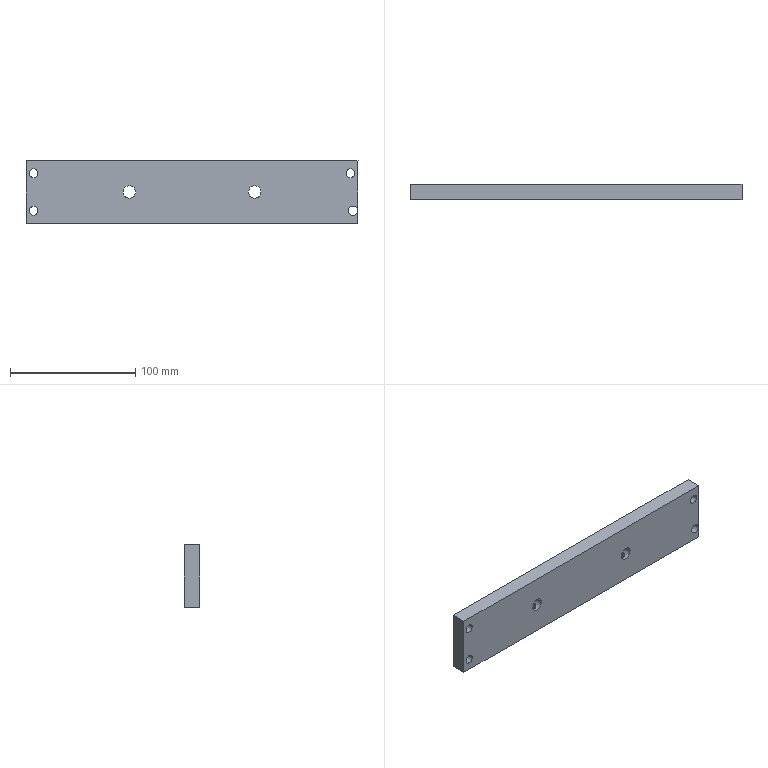Component | SolidWorks | AdjustmentTopPlate-1 | 1 solid | 22 faces | box 265 x 12 x 50 mm | volume 153730 mm3 | cylinder 16 | plane 6 | commonest cylinder face diameters 7 x6 6.8 x4 10 x4 7.46 x2
build123d program:
from build123d import *

# Parameters (mm, degrees)
SKETCH1_W             = 265
SKETCH1_H             = 50
SKETCH1_R             = 3.5
SKETCH1_R_2           = 3.73
EXTRUDE1_DEPTH        = 12
SKETCH2_R             = 5
EXTRUDE2_DEPTH        = 252.765
M8_TAPPED_HOLE1_D     = 6.8
M8_TAPPED_HOLE1_DEPTH = 22.25
M8_TAPPED_HOLE1_TIP   = 2.043


with BuildPart() as part:
    # Sketch1 → Extrude1 (new body)
    with BuildSketch(Plane.XY):
        with Locations((115.517, -16.583)):
            Rectangle(SKETCH1_W, SKETCH1_H)
        with Locations((-10.983, -1.583)):
            Circle(SKETCH1_R, mode=Mode.SUBTRACT)
        with Locations((242.017, -1.649)):
            Circle(SKETCH1_R, mode=Mode.SUBTRACT)
        with Locations((-10.983, -31.583)):
            Circle(SKETCH1_R, mode=Mode.SUBTRACT)
        with Locations((244.017, -31.583)):
            Circle(SKETCH1_R_2, mode=Mode.SUBTRACT)
    extrude(amount=EXTRUDE1_DEPTH)

    # Sketch2 → Extrude2 (cut, through all)
    with BuildSketch(Plane.XY.offset(12)):
        with Locations((65.517, -16.583)):
            Circle(SKETCH2_R)
        with Locations((165.517, -16.583)):
            Circle(SKETCH2_R)
    extrude(amount=-EXTRUDE2_DEPTH, mode=Mode.SUBTRACT)

    # M8 Tapped Hole1
    with Locations(Plane.XZ.offset(41.583)):
        with Locations((65.517, 6), (165.517, 6)):
            Hole(M8_TAPPED_HOLE1_D / 2, depth=M8_TAPPED_HOLE1_DEPTH)
            with Locations((0, 0, -(M8_TAPPED_HOLE1_DEPTH + M8_TAPPED_HOLE1_TIP / 2))):  # 118° drill point
                Cone(0, M8_TAPPED_HOLE1_D / 2, M8_TAPPED_HOLE1_TIP, mode=Mode.SUBTRACT)


solid = part.part

# Placed as in the assembly
solid = solid.moved(Location((-280.301, 717.983, -63.917), (90, 0, 0)))
STEP:
#1=CARTESIAN_POINT('',(-8.456,27.897,-3.366));
#2=VERTEX_POINT('',#1);
#3=CARTESIAN_POINT('',(-8.456,28.165,-3.366));
#4=VERTEX_POINT('',#3);
#5=CARTESIAN_POINT('',(-8.456,27.897,-3.366));
#6=CARTESIAN_POINT('',(-8.465,27.897,-3.366));
#7=CARTESIAN_POINT('',(-8.474,27.898,-3.366));
#8=CARTESIAN_POINT('',(-8.492,27.902,-3.363));
#9=CARTESIAN_POINT('',(-8.5,27.904,-3.361));
#10=CARTESIAN_POINT('',(-8.517,27.911,-3.357));
#11=CARTESIAN_POINT('',(-8.524,27.915,-3.354));
#12=CARTESIAN_POINT('',(-8.538,27.925,-3.348));
#13=CARTESIAN_POINT('',(-8.545,27.931,-3.345));
#14=CARTESIAN_POINT('',(-8.557,27.943,-3.338));
#15=CARTESIAN_POINT('',(-8.562,27.949,-3.335));
#16=CARTESIAN_POINT('',(-8.572,27.963,-3.329));
#17=CARTESIAN_POINT('',(-8.576,27.971,-3.325));
#18=CARTESIAN_POINT('',(-8.583,27.987,-3.32));
#19=CARTESIAN_POINT('',(-8.585,27.995,-3.318));
#20=CARTESIAN_POINT('',(-8.589,28.013,-3.314));
#21=CARTESIAN_POINT('',(-8.59,28.022,-3.314));
#22=CARTESIAN_POINT('',(-8.59,28.035,-3.314));
#23=CARTESIAN_POINT('',(-8.59,28.04,-3.314));
#24=CARTESIAN_POINT('',(-8.589,28.049,-3.315));
#25=CARTESIAN_POINT('',(-8.588,28.054,-3.315));
#26=CARTESIAN_POINT('',(-8.585,28.067,-3.318));
#27=CARTESIAN_POINT('',(-8.583,28.075,-3.32));
#28=CARTESIAN_POINT('',(-8.576,28.091,-3.326));
#29=CARTESIAN_POINT('',(-8.572,28.099,-3.329));
#30=CARTESIAN_POINT('',(-8.562,28.113,-3.335));
#31=CARTESIAN_POINT('',(-8.557,28.119,-3.338));
#32=CARTESIAN_POINT('',(-8.545,28.131,-3.345));
#33=CARTESIAN_POINT('',(-8.538,28.137,-3.348));
#34=CARTESIAN_POINT('',(-8.524,28.146,-3.354));
#35=CARTESIAN_POINT('',(-8.517,28.151,-3.357));
#36=CARTESIAN_POINT('',(-8.501,28.157,-3.361));
#37=CARTESIAN_POINT('',(-8.492,28.16,-3.363));
#38=CARTESIAN_POINT('',(-8.474,28.164,-3.366));
#39=CARTESIAN_POINT('',(-8.465,28.165,-3.366));
#40=CARTESIAN_POINT('',(-8.456,28.165,-3.366));
#41=B_SPLINE_CURVE_WITH_KNOTS('',3,(#5,#6,#7,#8,#9,#10,#11,#12,#13,#14,#15,#16,#17,#18,#19,#20,#21,#22,#23,#24,#25,#26,#27,#28,#29,#30,#31,#32,#33,#34,#35,#36,#37,#38,#39,#40),.UNSPECIFIED.,.F.,.F.,(4,2,2,2,2,2,2,2,2,2,2,2,2,2,2,2,2,4),(0.01101,0.0117,0.01239,0.01307,0.01376,0.01445,0.01513,0.01582,0.01651,0.01685,0.0172,0.01788,0.01857,0.01926,0.01995,0.02063,0.02132,0.02201),.UNSPECIFIED.);
#42=EDGE_CURVE('',#2,#4,#41,.T.);
#43=ORIENTED_EDGE('',*,*,#42,.F.);
#44=CARTESIAN_POINT('',(-8.456,27.897,-4.154));
#45=VERTEX_POINT('',#44);
#46=CARTESIAN_POINT('',(-8.456,27.897,-4.154));
#47=DIRECTION('',(-0.,-0.,-1.));
#48=VECTOR('',#47,39.37);
#49=LINE('',#46,#48);
#50=EDGE_CURVE('',#2,#45,#49,.T.);
#51=ORIENTED_EDGE('',*,*,#50,.T.);
#52=CARTESIAN_POINT('',(-8.456,28.165,-4.154));
#53=VERTEX_POINT('',#52);
#54=CARTESIAN_POINT('',(-8.456,28.031,-4.154));
#55=DIRECTION('',(-0.,-0.,-1.));
#56=DIRECTION('',(0.,1.,0.));
#57=AXIS2_PLACEMENT_3D('',#54,#55,#56);
#58=CIRCLE('',#57,0.1339);
#59=EDGE_CURVE('',#45,#53,#58,.T.);
#60=ORIENTED_EDGE('',*,*,#59,.T.);
#61=CARTESIAN_POINT('',(-8.456,28.165,-4.154));
#62=DIRECTION('',(-0.,-0.,-1.));
#63=VECTOR('',#62,39.37);
#64=LINE('',#61,#63);
#65=EDGE_CURVE('',#4,#53,#64,.T.);
#66=ORIENTED_EDGE('',*,*,#65,.F.);
#67=EDGE_LOOP('',(#43,#51,#60,#66));
#68=FACE_OUTER_BOUND('',#67,.T.);
#69=CARTESIAN_POINT('',(-8.456,28.031,-4.154));
#70=DIRECTION('',(-0.,-0.,-1.));
#71=DIRECTION('',(0.,1.,0.));
#72=AXIS2_PLACEMENT_3D('',#69,#70,#71);
#73=CYLINDRICAL_SURFACE('',#72,0.1339);
#74=ADVANCED_FACE('',(#68),#73,.F.);
#75=CARTESIAN_POINT('',(-4.519,27.897,-3.366));
#76=VERTEX_POINT('',#75);
#77=CARTESIAN_POINT('',(-4.519,28.165,-3.366));
#78=VERTEX_POINT('',#77);
#79=CARTESIAN_POINT('',(-4.519,27.897,-3.366));
#80=CARTESIAN_POINT('',(-4.528,27.897,-3.366));
#81=CARTESIAN_POINT('',(-4.537,27.898,-3.366));
#82=CARTESIAN_POINT('',(-4.555,27.902,-3.363));
#83=CARTESIAN_POINT('',(-4.563,27.904,-3.361));
#84=CARTESIAN_POINT('',(-4.58,27.911,-3.357));
#85=CARTESIAN_POINT('',(-4.587,27.915,-3.354));
#86=CARTESIAN_POINT('',(-4.601,27.925,-3.348));
#87=CARTESIAN_POINT('',(-4.608,27.931,-3.345));
#88=CARTESIAN_POINT('',(-4.62,27.943,-3.338));
#89=CARTESIAN_POINT('',(-4.625,27.949,-3.335));
#90=CARTESIAN_POINT('',(-4.635,27.963,-3.329));
#91=CARTESIAN_POINT('',(-4.639,27.971,-3.325));
#92=CARTESIAN_POINT('',(-4.646,27.987,-3.32));
#93=CARTESIAN_POINT('',(-4.648,27.995,-3.318));
#94=CARTESIAN_POINT('',(-4.652,28.013,-3.314));
#95=CARTESIAN_POINT('',(-4.653,28.022,-3.314));
#96=CARTESIAN_POINT('',(-4.653,28.035,-3.314));
#97=CARTESIAN_POINT('',(-4.653,28.04,-3.314));
#98=CARTESIAN_POINT('',(-4.652,28.049,-3.315));
#99=CARTESIAN_POINT('',(-4.651,28.054,-3.315));
#100=CARTESIAN_POINT('',(-4.648,28.067,-3.318));
#101=CARTESIAN_POINT('',(-4.646,28.075,-3.32));
#102=CARTESIAN_POINT('',(-4.639,28.091,-3.326));
#103=CARTESIAN_POINT('',(-4.635,28.099,-3.329));
#104=CARTESIAN_POINT('',(-4.625,28.113,-3.335));
#105=CARTESIAN_POINT('',(-4.62,28.119,-3.338));
#106=CARTESIAN_POINT('',(-4.608,28.131,-3.345));
#107=CARTESIAN_POINT('',(-4.601,28.137,-3.348));
#108=CARTESIAN_POINT('',(-4.587,28.146,-3.354));
#109=CARTESIAN_POINT('',(-4.58,28.151,-3.357));
#110=CARTESIAN_POINT('',(-4.564,28.157,-3.361));
#111=CARTESIAN_POINT('',(-4.555,28.16,-3.363));
#112=CARTESIAN_POINT('',(-4.537,28.164,-3.366));
#113=CARTESIAN_POINT('',(-4.528,28.165,-3.366));
#114=CARTESIAN_POINT('',(-4.519,28.165,-3.366));
#115=B_SPLINE_CURVE_WITH_KNOTS('',3,(#79,#80,#81,#82,#83,#84,#85,#86,#87,#88,#89,#90,#91,#92,#93,#94,#95,#96,#97,#98,#99,#100,#101,#102,#103,#104,#105,#106,#107,#108,#109,#110,#111,#112,#113,#114),.UNSPECIFIED.,.F.,.F.,(4,2,2,2,2,2,2,2,2,2,2,2,2,2,2,2,2,4),(0.01101,0.0117,0.01239,0.01307,0.01376,0.01445,0.01513,0.01582,0.01651,0.01685,0.0172,0.01788,0.01857,0.01926,0.01995,0.02063,0.02132,0.02201),.UNSPECIFIED.);
#116=EDGE_CURVE('',#76,#78,#115,.T.);
#117=ORIENTED_EDGE('',*,*,#116,.F.);
#118=CARTESIAN_POINT('',(-4.519,27.897,-4.154));
#119=VERTEX_POINT('',#118);
#120=CARTESIAN_POINT('',(-4.519,27.897,-4.154));
#121=DIRECTION('',(-0.,-0.,-1.));
#122=VECTOR('',#121,39.37);
#123=LINE('',#120,#122);
#124=EDGE_CURVE('',#76,#119,#123,.T.);
#125=ORIENTED_EDGE('',*,*,#124,.T.);
#126=CARTESIAN_POINT('',(-4.519,28.165,-4.154));
#127=VERTEX_POINT('',#126);
#128=CARTESIAN_POINT('',(-4.519,28.031,-4.154));
#129=DIRECTION('',(-0.,-0.,-1.));
#130=DIRECTION('',(0.,1.,0.));
#131=AXIS2_PLACEMENT_3D('',#128,#129,#130);
#132=CIRCLE('',#131,0.1339);
#133=EDGE_CURVE('',#119,#127,#132,.T.);
#134=ORIENTED_EDGE('',*,*,#133,.T.);
#135=CARTESIAN_POINT('',(-4.519,28.165,-4.154));
#136=DIRECTION('',(-0.,-0.,-1.));
#137=VECTOR('',#136,39.37);
#138=LINE('',#135,#137);
#139=EDGE_CURVE('',#78,#127,#138,.T.);
#140=ORIENTED_EDGE('',*,*,#139,.F.);
#141=EDGE_LOOP('',(#117,#125,#134,#140));
#142=FACE_OUTER_BOUND('',#141,.T.);
#143=CARTESIAN_POINT('',(-4.519,28.031,-4.154));
#144=DIRECTION('',(-0.,-0.,-1.));
#145=DIRECTION('',(0.,1.,0.));
#146=AXIS2_PLACEMENT_3D('',#143,#144,#145);
#147=CYLINDRICAL_SURFACE('',#146,0.1339);
#148=ADVANCED_FACE('',(#142),#147,.F.);
#149=CARTESIAN_POINT('',(-4.519,28.165,-3.366));
#150=CARTESIAN_POINT('',(-4.51,28.165,-3.366));
#151=CARTESIAN_POINT('',(-4.501,28.164,-3.366));
#152=CARTESIAN_POINT('',(-4.483,28.16,-3.363));
#153=CARTESIAN_POINT('',(-4.475,28.157,-3.361));
#154=CARTESIAN_POINT('',(-4.459,28.151,-3.357));
#155=CARTESIAN_POINT('',(-4.451,28.146,-3.354));
#156=CARTESIAN_POINT('',(-4.437,28.137,-3.348));
#157=CARTESIAN_POINT('',(-4.43,28.131,-3.345));
#158=CARTESIAN_POINT('',(-4.418,28.119,-3.338));
#159=CARTESIAN_POINT('',(-4.413,28.113,-3.335));
#160=CARTESIAN_POINT('',(-4.403,28.099,-3.329));
#161=CARTESIAN_POINT('',(-4.399,28.091,-3.326));
#162=CARTESIAN_POINT('',(-4.392,28.075,-3.32));
#163=CARTESIAN_POINT('',(-4.39,28.067,-3.318));
#164=CARTESIAN_POINT('',(-4.387,28.054,-3.315));
#165=CARTESIAN_POINT('',(-4.386,28.049,-3.315));
#166=CARTESIAN_POINT('',(-4.385,28.04,-3.314));
#167=CARTESIAN_POINT('',(-4.385,28.035,-3.314));
#168=CARTESIAN_POINT('',(-4.385,28.022,-3.314));
#169=CARTESIAN_POINT('',(-4.386,28.013,-3.314));
#170=CARTESIAN_POINT('',(-4.39,27.995,-3.318));
#171=CARTESIAN_POINT('',(-4.392,27.987,-3.32));
#172=CARTESIAN_POINT('',(-4.399,27.971,-3.325));
#173=CARTESIAN_POINT('',(-4.403,27.963,-3.329));
#174=CARTESIAN_POINT('',(-4.413,27.949,-3.335));
#175=CARTESIAN_POINT('',(-4.418,27.943,-3.338));
#176=CARTESIAN_POINT('',(-4.436,27.924,-3.348));
#177=CARTESIAN_POINT('',(-4.45,27.915,-3.354));
#178=CARTESIAN_POINT('',(-4.475,27.904,-3.361));
#179=CARTESIAN_POINT('',(-4.483,27.902,-3.363));
#180=CARTESIAN_POINT('',(-4.501,27.898,-3.365));
#181=CARTESIAN_POINT('',(-4.51,27.897,-3.366));
#182=CARTESIAN_POINT('',(-4.519,27.897,-3.366));
#183=B_SPLINE_CURVE_WITH_KNOTS('',3,(#149,#150,#151,#152,#153,#154,#155,#156,#157,#158,#159,#160,#161,#162,#163,#164,#165,#166,#167,#168,#169,#170,#171,#172,#173,#174,#175,#176,#177,#178,#179,#180,#181,#182),.UNSPECIFIED.,.F.,.F.,(4,2,2,2,2,2,2,2,2,2,2,2,2,2,2,2,4),(0.,0.0006882,0.001376,0.002065,0.002753,0.003441,0.004129,0.004818,0.005162,0.005506,0.006194,0.006882,0.007571,0.008259,0.009635,0.01032,0.01101),.UNSPECIFIED.);
#184=EDGE_CURVE('',#78,#76,#183,.T.);
#185=ORIENTED_EDGE('',*,*,#184,.T.);
#186=ORIENTED_EDGE('',*,*,#116,.T.);
#187=EDGE_LOOP('',(#185,#186));
#188=FACE_BOUND('',#187,.T.);
#189=CARTESIAN_POINT('',(-4.716,28.267,-3.169));
#190=VERTEX_POINT('',#189);
#191=CARTESIAN_POINT('',(-4.322,28.267,-3.169));
#192=VERTEX_POINT('',#191);
#193=CARTESIAN_POINT('',(-4.519,28.267,-3.169));
#194=DIRECTION('',(0.,-1.,0.));
#195=DIRECTION('',(1.,0.,-0.));
#196=AXIS2_PLACEMENT_3D('',#193,#194,#195);
#197=CIRCLE('',#196,0.1969);
#198=EDGE_CURVE('',#190,#192,#197,.T.);
#199=ORIENTED_EDGE('',*,*,#198,.F.);
#200=CARTESIAN_POINT('',(-4.716,27.795,-3.169));
#201=VERTEX_POINT('',#200);
#202=CARTESIAN_POINT('',(-4.716,28.267,-3.169));
#203=DIRECTION('',(0.,-1.,0.));
#204=VECTOR('',#203,39.37);
#205=LINE('',#202,#204);
#206=EDGE_CURVE('',#190,#201,#205,.T.);
#207=ORIENTED_EDGE('',*,*,#206,.T.);
#208=CARTESIAN_POINT('',(-4.322,27.795,-3.169));
#209=VERTEX_POINT('',#208);
#210=CARTESIAN_POINT('',(-4.519,27.795,-3.169));
#211=DIRECTION('',(0.,-1.,0.));
#212=DIRECTION('',(1.,0.,-0.));
#213=AXIS2_PLACEMENT_3D('',#210,#211,#212);
#214=CIRCLE('',#213,0.1969);
#215=EDGE_CURVE('',#201,#209,#214,.T.);
#216=ORIENTED_EDGE('',*,*,#215,.T.);
#217=CARTESIAN_POINT('',(-4.322,28.267,-3.169));
#218=DIRECTION('',(0.,-1.,0.));
#219=VECTOR('',#218,39.37);
#220=LINE('',#217,#219);
#221=EDGE_CURVE('',#192,#209,#220,.T.);
#222=ORIENTED_EDGE('',*,*,#221,.F.);
#223=EDGE_LOOP('',(#199,#207,#216,#222));
#224=FACE_OUTER_BOUND('',#223,.T.);
#225=CARTESIAN_POINT('',(-4.519,28.267,-3.169));
#226=DIRECTION('',(0.,-1.,0.));
#227=DIRECTION('',(1.,0.,-0.));
#228=AXIS2_PLACEMENT_3D('',#225,#226,#227);
#229=CYLINDRICAL_SURFACE('',#228,0.1969);
#230=ADVANCED_FACE('',(#188,#224),#229,.F.);
#231=CARTESIAN_POINT('',(-8.456,28.165,-3.366));
#232=CARTESIAN_POINT('',(-8.447,28.165,-3.366));
#233=CARTESIAN_POINT('',(-8.438,28.164,-3.366));
#234=CARTESIAN_POINT('',(-8.42,28.16,-3.363));
#235=CARTESIAN_POINT('',(-8.412,28.157,-3.361));
#236=CARTESIAN_POINT('',(-8.396,28.151,-3.357));
#237=CARTESIAN_POINT('',(-8.388,28.146,-3.354));
#238=CARTESIAN_POINT('',(-8.374,28.137,-3.348));
#239=CARTESIAN_POINT('',(-8.367,28.131,-3.345));
#240=CARTESIAN_POINT('',(-8.355,28.119,-3.338));
#241=CARTESIAN_POINT('',(-8.35,28.113,-3.335));
#242=CARTESIAN_POINT('',(-8.34,28.099,-3.329));
#243=CARTESIAN_POINT('',(-8.336,28.091,-3.326));
#244=CARTESIAN_POINT('',(-8.329,28.075,-3.32));
#245=CARTESIAN_POINT('',(-8.327,28.067,-3.318));
#246=CARTESIAN_POINT('',(-8.324,28.054,-3.315));
#247=CARTESIAN_POINT('',(-8.323,28.049,-3.315));
#248=CARTESIAN_POINT('',(-8.322,28.04,-3.314));
#249=CARTESIAN_POINT('',(-8.322,28.035,-3.314));
#250=CARTESIAN_POINT('',(-8.322,28.022,-3.314));
#251=CARTESIAN_POINT('',(-8.323,28.013,-3.314));
#252=CARTESIAN_POINT('',(-8.327,27.995,-3.318));
#253=CARTESIAN_POINT('',(-8.329,27.987,-3.32));
#254=CARTESIAN_POINT('',(-8.336,27.971,-3.325));
#255=CARTESIAN_POINT('',(-8.34,27.963,-3.329));
#256=CARTESIAN_POINT('',(-8.35,27.949,-3.335));
#257=CARTESIAN_POINT('',(-8.355,27.943,-3.338));
#258=CARTESIAN_POINT('',(-8.373,27.924,-3.348));
#259=CARTESIAN_POINT('',(-8.387,27.915,-3.354));
#260=CARTESIAN_POINT('',(-8.412,27.904,-3.361));
#261=CARTESIAN_POINT('',(-8.42,27.902,-3.363));
#262=CARTESIAN_POINT('',(-8.438,27.898,-3.365));
#263=CARTESIAN_POINT('',(-8.447,27.897,-3.366));
#264=CARTESIAN_POINT('',(-8.456,27.897,-3.366));
#265=B_SPLINE_CURVE_WITH_KNOTS('',3,(#231,#232,#233,#234,#235,#236,#237,#238,#239,#240,#241,#242,#243,#244,#245,#246,#247,#248,#249,#250,#251,#252,#253,#254,#255,#256,#257,#258,#259,#260,#261,#262,#263,#264),.UNSPECIFIED.,.F.,.F.,(4,2,2,2,2,2,2,2,2,2,2,2,2,2,2,2,4),(0.,0.0006882,0.001376,0.002065,0.002753,0.003441,0.004129,0.004818,0.005162,0.005506,0.006194,0.006882,0.007571,0.008259,0.009635,0.01032,0.01101),.UNSPECIFIED.);
#266=EDGE_CURVE('',#4,#2,#265,.T.);
#267=ORIENTED_EDGE('',*,*,#266,.T.);
#268=ORIENTED_EDGE('',*,*,#42,.T.);
#269=EDGE_LOOP('',(#267,#268));
#270=FACE_BOUND('',#269,.T.);
#271=CARTESIAN_POINT('',(-8.653,28.267,-3.169));
#272=VERTEX_POINT('',#271);
#273=CARTESIAN_POINT('',(-8.259,28.267,-3.169));
#274=VERTEX_POINT('',#273);
#275=CARTESIAN_POINT('',(-8.456,28.267,-3.169));
#276=DIRECTION('',(0.,-1.,0.));
#277=DIRECTION('',(1.,0.,-0.));
#278=AXIS2_PLACEMENT_3D('',#275,#276,#277);
#279=CIRCLE('',#278,0.1969);
#280=EDGE_CURVE('',#272,#274,#279,.T.);
#281=ORIENTED_EDGE('',*,*,#280,.F.);
#282=CARTESIAN_POINT('',(-8.653,27.795,-3.169));
#283=VERTEX_POINT('',#282);
#284=CARTESIAN_POINT('',(-8.653,28.267,-3.169));
#285=DIRECTION('',(0.,-1.,0.));
#286=VECTOR('',#285,39.37);
#287=LINE('',#284,#286);
#288=EDGE_CURVE('',#272,#283,#287,.T.);
#289=ORIENTED_EDGE('',*,*,#288,.T.);
#290=CARTESIAN_POINT('',(-8.259,27.795,-3.169));
#291=VERTEX_POINT('',#290);
#292=CARTESIAN_POINT('',(-8.456,27.795,-3.169));
#293=DIRECTION('',(0.,-1.,0.));
#294=DIRECTION('',(1.,0.,-0.));
#295=AXIS2_PLACEMENT_3D('',#292,#293,#294);
#296=CIRCLE('',#295,0.1969);
#297=EDGE_CURVE('',#283,#291,#296,.T.);
#298=ORIENTED_EDGE('',*,*,#297,.T.);
#299=CARTESIAN_POINT('',(-8.259,28.267,-3.169));
#300=DIRECTION('',(0.,-1.,0.));
#301=VECTOR('',#300,39.37);
#302=LINE('',#299,#301);
#303=EDGE_CURVE('',#274,#291,#302,.T.);
#304=ORIENTED_EDGE('',*,*,#303,.F.);
#305=EDGE_LOOP('',(#281,#289,#298,#304));
#306=FACE_OUTER_BOUND('',#305,.T.);
#307=CARTESIAN_POINT('',(-8.456,28.267,-3.169));
#308=DIRECTION('',(0.,-1.,0.));
#309=DIRECTION('',(1.,0.,-0.));
#310=AXIS2_PLACEMENT_3D('',#307,#308,#309);
#311=CYLINDRICAL_SURFACE('',#310,0.1969);
#312=ADVANCED_FACE('',(#270,#306),#311,.F.);
#313=CARTESIAN_POINT('',(-1.575,27.795,-3.76));
#314=VERTEX_POINT('',#313);
#315=CARTESIAN_POINT('',(-1.282,27.795,-3.76));
#316=VERTEX_POINT('',#315);
#317=CARTESIAN_POINT('',(-1.428,27.795,-3.76));
#318=DIRECTION('',(0.,-1.,0.));
#319=DIRECTION('',(1.,0.,-0.));
#320=AXIS2_PLACEMENT_3D('',#317,#318,#319);
#321=CIRCLE('',#320,0.1469);
#322=EDGE_CURVE('',#314,#316,#321,.T.);
#323=ORIENTED_EDGE('',*,*,#322,.T.);
#324=CARTESIAN_POINT('',(-1.282,28.267,-3.76));
#325=VERTEX_POINT('',#324);
#326=CARTESIAN_POINT('',(-1.282,27.795,-3.76));
#327=DIRECTION('',(-0.,1.,-0.));
#328=VECTOR('',#327,39.37);
#329=LINE('',#326,#328);
#330=EDGE_CURVE('',#316,#325,#329,.T.);
#331=ORIENTED_EDGE('',*,*,#330,.T.);
#332=CARTESIAN_POINT('',(-1.575,28.267,-3.76));
#333=VERTEX_POINT('',#332);
#334=CARTESIAN_POINT('',(-1.428,28.267,-3.76));
#335=DIRECTION('',(0.,-1.,0.));
#336=DIRECTION('',(1.,0.,-0.));
#337=AXIS2_PLACEMENT_3D('',#334,#335,#336);
#338=CIRCLE('',#337,0.1469);
#339=EDGE_CURVE('',#333,#325,#338,.T.);
#340=ORIENTED_EDGE('',*,*,#339,.F.);
#341=CARTESIAN_POINT('',(-1.575,27.795,-3.76));
#342=DIRECTION('',(-0.,1.,-0.));
#343=VECTOR('',#342,39.37);
#344=LINE('',#341,#343);
#345=EDGE_CURVE('',#314,#333,#344,.T.);
#346=ORIENTED_EDGE('',*,*,#345,.F.);
#347=EDGE_LOOP('',(#323,#331,#340,#346));
#348=FACE_OUTER_BOUND('',#347,.T.);
#349=CARTESIAN_POINT('',(-1.428,27.795,-3.76));
#350=DIRECTION('',(-0.,1.,-0.));
#351=DIRECTION('',(-1.,0.,0.));
#352=AXIS2_PLACEMENT_3D('',#349,#350,#351);
#353=CYLINDRICAL_SURFACE('',#352,0.1469);
#354=ADVANCED_FACE('',(#348),#353,.F.);
#355=CARTESIAN_POINT('',(-1.645,27.795,-2.581));
#356=VERTEX_POINT('',#355);
#357=CARTESIAN_POINT('',(-1.369,27.795,-2.581));
#358=VERTEX_POINT('',#357);
#359=CARTESIAN_POINT('',(-1.507,27.795,-2.581));
#360=DIRECTION('',(0.,-1.,0.));
#361=DIRECTION('',(1.,0.,-0.));
#362=AXIS2_PLACEMENT_3D('',#359,#360,#361);
#363=CIRCLE('',#362,0.1378);
#364=EDGE_CURVE('',#356,#358,#363,.T.);
#365=ORIENTED_EDGE('',*,*,#364,.T.);
#366=CARTESIAN_POINT('',(-1.369,28.267,-2.581));
#367=VERTEX_POINT('',#366);
#368=CARTESIAN_POINT('',(-1.369,27.795,-2.581));
#369=DIRECTION('',(-0.,1.,-0.));
#370=VECTOR('',#369,39.37);
#371=LINE('',#368,#370);
#372=EDGE_CURVE('',#358,#367,#371,.T.);
#373=ORIENTED_EDGE('',*,*,#372,.T.);
#374=CARTESIAN_POINT('',(-1.645,28.267,-2.581));
#375=VERTEX_POINT('',#374);
#376=CARTESIAN_POINT('',(-1.507,28.267,-2.581));
#377=DIRECTION('',(0.,-1.,0.));
#378=DIRECTION('',(1.,0.,-0.));
#379=AXIS2_PLACEMENT_3D('',#376,#377,#378);
#380=CIRCLE('',#379,0.1378);
#381=EDGE_CURVE('',#375,#367,#380,.T.);
#382=ORIENTED_EDGE('',*,*,#381,.F.);
#383=CARTESIAN_POINT('',(-1.645,27.795,-2.581));
#384=DIRECTION('',(-0.,1.,-0.));
#385=VECTOR('',#384,39.37);
#386=LINE('',#383,#385);
#387=EDGE_CURVE('',#356,#375,#386,.T.);
#388=ORIENTED_EDGE('',*,*,#387,.F.);
#389=EDGE_LOOP('',(#365,#373,#382,#388));
#390=FACE_OUTER_BOUND('',#389,.T.);
#391=CARTESIAN_POINT('',(-1.507,27.795,-2.581));
#392=DIRECTION('',(-0.,1.,-0.));
#393=DIRECTION('',(-1.,0.,0.));
#394=AXIS2_PLACEMENT_3D('',#391,#392,#393);
#395=CYLINDRICAL_SURFACE('',#394,0.1378);
#396=ADVANCED_FACE('',(#390),#395,.F.);
#397=CARTESIAN_POINT('',(-11.606,27.795,-2.579));
#398=VERTEX_POINT('',#397);
#399=CARTESIAN_POINT('',(-11.33,27.795,-2.579));
#400=VERTEX_POINT('',#399);
#401=CARTESIAN_POINT('',(-11.468,27.795,-2.579));
#402=DIRECTION('',(0.,-1.,0.));
#403=DIRECTION('',(1.,0.,-0.));
#404=AXIS2_PLACEMENT_3D('',#401,#402,#403);
#405=CIRCLE('',#404,0.1378);
#406=EDGE_CURVE('',#398,#400,#405,.T.);
#407=ORIENTED_EDGE('',*,*,#406,.T.);
#408=CARTESIAN_POINT('',(-11.33,28.267,-2.579));
#409=VERTEX_POINT('',#408);
#410=CARTESIAN_POINT('',(-11.33,27.795,-2.579));
#411=DIRECTION('',(-0.,1.,-0.));
#412=VECTOR('',#411,39.37);
#413=LINE('',#410,#412);
#414=EDGE_CURVE('',#400,#409,#413,.T.);
#415=ORIENTED_EDGE('',*,*,#414,.T.);
#416=CARTESIAN_POINT('',(-11.606,28.267,-2.579));
#417=VERTEX_POINT('',#416);
#418=CARTESIAN_POINT('',(-11.468,28.267,-2.579));
#419=DIRECTION('',(0.,-1.,0.));
#420=DIRECTION('',(1.,0.,-0.));
#421=AXIS2_PLACEMENT_3D('',#418,#419,#420);
#422=CIRCLE('',#421,0.1378);
#423=EDGE_CURVE('',#417,#409,#422,.T.);
#424=ORIENTED_EDGE('',*,*,#423,.F.);
#425=CARTESIAN_POINT('',(-11.606,27.795,-2.579));
#426=DIRECTION('',(-0.,1.,-0.));
#427=VECTOR('',#426,39.37);
#428=LINE('',#425,#427);
#429=EDGE_CURVE('',#398,#417,#428,.T.);
#430=ORIENTED_EDGE('',*,*,#429,.F.);
#431=EDGE_LOOP('',(#407,#415,#424,#430));
#432=FACE_OUTER_BOUND('',#431,.T.);
#433=CARTESIAN_POINT('',(-11.468,27.795,-2.579));
#434=DIRECTION('',(-0.,1.,-0.));
#435=DIRECTION('',(-1.,0.,0.));
#436=AXIS2_PLACEMENT_3D('',#433,#434,#435);
#437=CYLINDRICAL_SURFACE('',#436,0.1378);
#438=ADVANCED_FACE('',(#432),#437,.F.);
#439=CARTESIAN_POINT('',(-11.606,27.795,-3.76));
#440=VERTEX_POINT('',#439);
#441=CARTESIAN_POINT('',(-11.33,27.795,-3.76));
#442=VERTEX_POINT('',#441);
#443=CARTESIAN_POINT('',(-11.468,27.795,-3.76));
#444=DIRECTION('',(0.,-1.,0.));
#445=DIRECTION('',(1.,0.,-0.));
#446=AXIS2_PLACEMENT_3D('',#443,#444,#445);
#447=CIRCLE('',#446,0.1378);
#448=EDGE_CURVE('',#440,#442,#447,.T.);
#449=ORIENTED_EDGE('',*,*,#448,.T.);
#450=CARTESIAN_POINT('',(-11.33,28.267,-3.76));
#451=VERTEX_POINT('',#450);
#452=CARTESIAN_POINT('',(-11.33,27.795,-3.76));
#453=DIRECTION('',(-0.,1.,-0.));
#454=VECTOR('',#453,39.37);
#455=LINE('',#452,#454);
#456=EDGE_CURVE('',#442,#451,#455,.T.);
#457=ORIENTED_EDGE('',*,*,#456,.T.);
#458=CARTESIAN_POINT('',(-11.606,28.267,-3.76));
#459=VERTEX_POINT('',#458);
#460=CARTESIAN_POINT('',(-11.468,28.267,-3.76));
#461=DIRECTION('',(0.,-1.,0.));
#462=DIRECTION('',(1.,0.,-0.));
#463=AXIS2_PLACEMENT_3D('',#460,#461,#462);
#464=CIRCLE('',#463,0.1378);
#465=EDGE_CURVE('',#459,#451,#464,.T.);
#466=ORIENTED_EDGE('',*,*,#465,.F.);
#467=CARTESIAN_POINT('',(-11.606,27.795,-3.76));
#468=DIRECTION('',(-0.,1.,-0.));
#469=VECTOR('',#468,39.37);
#470=LINE('',#467,#469);
#471=EDGE_CURVE('',#440,#459,#470,.T.);
#472=ORIENTED_EDGE('',*,*,#471,.F.);
#473=EDGE_LOOP('',(#449,#457,#466,#472));
#474=FACE_OUTER_BOUND('',#473,.T.);
#475=CARTESIAN_POINT('',(-11.468,27.795,-3.76));
#476=DIRECTION('',(-0.,1.,-0.));
#477=DIRECTION('',(-1.,0.,0.));
#478=AXIS2_PLACEMENT_3D('',#475,#476,#477);
#479=CYLINDRICAL_SURFACE('',#478,0.1378);
#480=ADVANCED_FACE('',(#474),#479,.F.);
#481=CARTESIAN_POINT('',(-4.519,27.795,-3.169));
#482=DIRECTION('',(0.,-1.,0.));
#483=DIRECTION('',(1.,0.,-0.));
#484=AXIS2_PLACEMENT_3D('',#481,#482,#483);
#485=CIRCLE('',#484,0.1969);
#486=EDGE_CURVE('',#209,#201,#485,.T.);
#487=ORIENTED_EDGE('',*,*,#486,.F.);
#488=ORIENTED_EDGE('',*,*,#215,.F.);
#489=EDGE_LOOP('',(#487,#488));
#490=FACE_BOUND('',#489,.T.);
#491=CARTESIAN_POINT('',(-8.456,27.795,-3.169));
#492=DIRECTION('',(0.,-1.,0.));
#493=DIRECTION('',(1.,0.,-0.));
#494=AXIS2_PLACEMENT_3D('',#491,#492,#493);
#495=CIRCLE('',#494,0.1969);
#496=EDGE_CURVE('',#291,#283,#495,.T.);
#497=ORIENTED_EDGE('',*,*,#496,.F.);
#498=ORIENTED_EDGE('',*,*,#297,.F.);
#499=EDGE_LOOP('',(#497,#498));
#500=FACE_BOUND('',#499,.T.);
#501=ORIENTED_EDGE('',*,*,#364,.F.);
#502=CARTESIAN_POINT('',(-1.507,27.795,-2.581));
#503=DIRECTION('',(0.,-1.,0.));
#504=DIRECTION('',(1.,0.,-0.));
#505=AXIS2_PLACEMENT_3D('',#502,#503,#504);
#506=CIRCLE('',#505,0.1378);
#507=EDGE_CURVE('',#358,#356,#506,.T.);
#508=ORIENTED_EDGE('',*,*,#507,.F.);
#509=EDGE_LOOP('',(#501,#508));
#510=FACE_BOUND('',#509,.T.);
#511=ORIENTED_EDGE('',*,*,#448,.F.);
#512=CARTESIAN_POINT('',(-11.468,27.795,-3.76));
#513=DIRECTION('',(0.,-1.,0.));
#514=DIRECTION('',(1.,0.,-0.));
#515=AXIS2_PLACEMENT_3D('',#512,#513,#514);
#516=CIRCLE('',#515,0.1378);
#517=EDGE_CURVE('',#442,#440,#516,.T.);
#518=ORIENTED_EDGE('',*,*,#517,.F.);
#519=EDGE_LOOP('',(#511,#518));
#520=FACE_BOUND('',#519,.T.);
#521=CARTESIAN_POINT('',(-11.704,27.795,-2.185));
#522=VERTEX_POINT('',#521);
#523=CARTESIAN_POINT('',(-11.704,27.795,-4.154));
#524=VERTEX_POINT('',#523);
#525=CARTESIAN_POINT('',(-11.704,27.795,-2.185));
#526=DIRECTION('',(-0.,-0.,-1.));
#527=VECTOR('',#526,39.37);
#528=LINE('',#525,#527);
#529=EDGE_CURVE('',#522,#524,#528,.T.);
#530=ORIENTED_EDGE('',*,*,#529,.T.);
#531=CARTESIAN_POINT('',(-1.271,27.795,-4.154));
#532=VERTEX_POINT('',#531);
#533=CARTESIAN_POINT('',(-11.704,27.795,-4.154));
#534=DIRECTION('',(1.,0.,-0.));
#535=VECTOR('',#534,39.37);
#536=LINE('',#533,#535);
#537=EDGE_CURVE('',#524,#532,#536,.T.);
#538=ORIENTED_EDGE('',*,*,#537,.T.);
#539=CARTESIAN_POINT('',(-1.271,27.795,-2.185));
#540=VERTEX_POINT('',#539);
#541=CARTESIAN_POINT('',(-1.271,27.795,-2.185));
#542=DIRECTION('',(0.,0.,1.));
#543=VECTOR('',#542,39.37);
#544=LINE('',#541,#543);
#545=EDGE_CURVE('',#532,#540,#544,.T.);
#546=ORIENTED_EDGE('',*,*,#545,.T.);
#547=CARTESIAN_POINT('',(-11.704,27.795,-2.185));
#548=DIRECTION('',(-1.,-0.,0.));
#549=VECTOR('',#548,39.37);
#550=LINE('',#547,#549);
#551=EDGE_CURVE('',#540,#522,#550,.T.);
#552=ORIENTED_EDGE('',*,*,#551,.T.);
#553=EDGE_LOOP('',(#530,#538,#546,#552));
#554=FACE_OUTER_BOUND('',#553,.T.);
#555=ORIENTED_EDGE('',*,*,#406,.F.);
#556=CARTESIAN_POINT('',(-11.468,27.795,-2.579));
#557=DIRECTION('',(0.,-1.,0.));
#558=DIRECTION('',(1.,0.,-0.));
#559=AXIS2_PLACEMENT_3D('',#556,#557,#558);
#560=CIRCLE('',#559,0.1378);
#561=EDGE_CURVE('',#400,#398,#560,.T.);
#562=ORIENTED_EDGE('',*,*,#561,.F.);
#563=EDGE_LOOP('',(#555,#562));
#564=FACE_BOUND('',#563,.T.);
#565=ORIENTED_EDGE('',*,*,#322,.F.);
#566=CARTESIAN_POINT('',(-1.428,27.795,-3.76));
#567=DIRECTION('',(0.,-1.,0.));
#568=DIRECTION('',(1.,0.,-0.));
#569=AXIS2_PLACEMENT_3D('',#566,#567,#568);
#570=CIRCLE('',#569,0.1469);
#571=EDGE_CURVE('',#316,#314,#570,.T.);
#572=ORIENTED_EDGE('',*,*,#571,.F.);
#573=EDGE_LOOP('',(#565,#572));
#574=FACE_BOUND('',#573,.T.);
#575=CARTESIAN_POINT('',(-11.704,27.795,-4.154));
#576=DIRECTION('',(0.,-1.,0.));
#577=DIRECTION('',(1.,0.,-0.));
#578=AXIS2_PLACEMENT_3D('',#575,#576,#577);
#579=PLANE('',#578);
#580=ADVANCED_FACE('',(#490,#500,#510,#520,#554,#564,#574),#579,.T.);
#581=CARTESIAN_POINT('',(-4.519,28.267,-3.169));
#582=DIRECTION('',(0.,-1.,0.));
#583=DIRECTION('',(1.,0.,-0.));
#584=AXIS2_PLACEMENT_3D('',#581,#582,#583);
#585=CIRCLE('',#584,0.1969);
#586=EDGE_CURVE('',#192,#190,#585,.T.);
#587=ORIENTED_EDGE('',*,*,#586,.T.);
#588=ORIENTED_EDGE('',*,*,#198,.T.);
#589=EDGE_LOOP('',(#587,#588));
#590=FACE_BOUND('',#589,.T.);
#591=CARTESIAN_POINT('',(-8.456,28.267,-3.169));
#592=DIRECTION('',(0.,-1.,0.));
#593=DIRECTION('',(1.,0.,-0.));
#594=AXIS2_PLACEMENT_3D('',#591,#592,#593);
#595=CIRCLE('',#594,0.1969);
#596=EDGE_CURVE('',#274,#272,#595,.T.);
#597=ORIENTED_EDGE('',*,*,#596,.T.);
#598=ORIENTED_EDGE('',*,*,#280,.T.);
#599=EDGE_LOOP('',(#597,#598));
#600=FACE_BOUND('',#599,.T.);
#601=CARTESIAN_POINT('',(-11.704,28.267,-2.185));
#602=VERTEX_POINT('',#601);
#603=CARTESIAN_POINT('',(-11.704,28.267,-4.154));
#604=VERTEX_POINT('',#603);
#605=CARTESIAN_POINT('',(-11.704,28.267,-2.185));
#606=DIRECTION('',(-0.,-0.,-1.));
#607=VECTOR('',#606,39.37);
#608=LINE('',#605,#607);
#609=EDGE_CURVE('',#602,#604,#608,.T.);
#610=ORIENTED_EDGE('',*,*,#609,.F.);
#611=CARTESIAN_POINT('',(-1.271,28.267,-2.185));
#612=VERTEX_POINT('',#611);
#613=CARTESIAN_POINT('',(-11.704,28.267,-2.185));
#614=DIRECTION('',(-1.,-0.,0.));
#615=VECTOR('',#614,39.37);
#616=LINE('',#613,#615);
#617=EDGE_CURVE('',#612,#602,#616,.T.);
#618=ORIENTED_EDGE('',*,*,#617,.F.);
#619=CARTESIAN_POINT('',(-1.271,28.267,-4.154));
#620=VERTEX_POINT('',#619);
#621=CARTESIAN_POINT('',(-1.271,28.267,-2.185));
#622=DIRECTION('',(0.,0.,1.));
#623=VECTOR('',#622,39.37);
#624=LINE('',#621,#623);
#625=EDGE_CURVE('',#620,#612,#624,.T.);
#626=ORIENTED_EDGE('',*,*,#625,.F.);
#627=CARTESIAN_POINT('',(-11.704,28.267,-4.154));
#628=DIRECTION('',(1.,0.,-0.));
#629=VECTOR('',#628,39.37);
#630=LINE('',#627,#629);
#631=EDGE_CURVE('',#604,#620,#630,.T.);
#632=ORIENTED_EDGE('',*,*,#631,.F.);
#633=EDGE_LOOP('',(#610,#618,#626,#632));
#634=FACE_OUTER_BOUND('',#633,.T.);
#635=ORIENTED_EDGE('',*,*,#465,.T.);
#636=CARTESIAN_POINT('',(-11.468,28.267,-3.76));
#637=DIRECTION('',(0.,-1.,0.));
#638=DIRECTION('',(1.,0.,-0.));
#639=AXIS2_PLACEMENT_3D('',#636,#637,#638);
#640=CIRCLE('',#639,0.1378);
#641=EDGE_CURVE('',#451,#459,#640,.T.);
#642=ORIENTED_EDGE('',*,*,#641,.T.);
#643=EDGE_LOOP('',(#635,#642));
#644=FACE_BOUND('',#643,.T.);
#645=ORIENTED_EDGE('',*,*,#423,.T.);
#646=CARTESIAN_POINT('',(-11.468,28.267,-2.579));
#647=DIRECTION('',(0.,-1.,0.));
#648=DIRECTION('',(1.,0.,-0.));
#649=AXIS2_PLACEMENT_3D('',#646,#647,#648);
#650=CIRCLE('',#649,0.1378);
#651=EDGE_CURVE('',#409,#417,#650,.T.);
#652=ORIENTED_EDGE('',*,*,#651,.T.);
#653=EDGE_LOOP('',(#645,#652));
#654=FACE_BOUND('',#653,.T.);
#655=ORIENTED_EDGE('',*,*,#381,.T.);
#656=CARTESIAN_POINT('',(-1.507,28.267,-2.581));
#657=DIRECTION('',(0.,-1.,0.));
#658=DIRECTION('',(1.,0.,-0.));
#659=AXIS2_PLACEMENT_3D('',#656,#657,#658);
#660=CIRCLE('',#659,0.1378);
#661=EDGE_CURVE('',#367,#375,#660,.T.);
#662=ORIENTED_EDGE('',*,*,#661,.T.);
#663=EDGE_LOOP('',(#655,#662));
#664=FACE_BOUND('',#663,.T.);
#665=ORIENTED_EDGE('',*,*,#339,.T.);
#666=CARTESIAN_POINT('',(-1.428,28.267,-3.76));
#667=DIRECTION('',(0.,-1.,0.));
#668=DIRECTION('',(1.,0.,-0.));
#669=AXIS2_PLACEMENT_3D('',#666,#667,#668);
#670=CIRCLE('',#669,0.1469);
#671=EDGE_CURVE('',#325,#333,#670,.T.);
#672=ORIENTED_EDGE('',*,*,#671,.T.);
#673=EDGE_LOOP('',(#665,#672));
#674=FACE_BOUND('',#673,.T.);
#675=CARTESIAN_POINT('',(-11.704,28.267,-4.154));
#676=DIRECTION('',(0.,-1.,0.));
#677=DIRECTION('',(1.,0.,-0.));
#678=AXIS2_PLACEMENT_3D('',#675,#676,#677);
#679=PLANE('',#678);
#680=ADVANCED_FACE('',(#590,#600,#634,#644,#654,#664,#674),#679,.F.);
#681=ORIENTED_EDGE('',*,*,#609,.T.);
#682=CARTESIAN_POINT('',(-11.704,27.795,-4.154));
#683=DIRECTION('',(-0.,1.,-0.));
#684=VECTOR('',#683,39.37);
#685=LINE('',#682,#684);
#686=EDGE_CURVE('',#524,#604,#685,.T.);
#687=ORIENTED_EDGE('',*,*,#686,.F.);
#688=ORIENTED_EDGE('',*,*,#529,.F.);
#689=CARTESIAN_POINT('',(-11.704,27.795,-2.185));
#690=DIRECTION('',(-0.,1.,-0.));
#691=VECTOR('',#690,39.37);
#692=LINE('',#689,#691);
#693=EDGE_CURVE('',#522,#602,#692,.T.);
#694=ORIENTED_EDGE('',*,*,#693,.T.);
#695=EDGE_LOOP('',(#681,#687,#688,#694));
#696=FACE_OUTER_BOUND('',#695,.T.);
#697=CARTESIAN_POINT('',(-11.704,27.795,-2.185));
#698=DIRECTION('',(1.,0.,-0.));
#699=DIRECTION('',(0.,0.,1.));
#700=AXIS2_PLACEMENT_3D('',#697,#698,#699);
#701=PLANE('',#700);
#702=ADVANCED_FACE('',(#696),#701,.F.);
#703=CARTESIAN_POINT('',(-8.456,28.031,-4.154));
#704=DIRECTION('',(-0.,-0.,-1.));
#705=DIRECTION('',(0.,1.,0.));
#706=AXIS2_PLACEMENT_3D('',#703,#704,#705);
#707=CIRCLE('',#706,0.1339);
#708=EDGE_CURVE('',#53,#45,#707,.T.);
#709=ORIENTED_EDGE('',*,*,#708,.F.);
#710=ORIENTED_EDGE('',*,*,#59,.F.);
#711=EDGE_LOOP('',(#709,#710));
#712=FACE_BOUND('',#711,.T.);
#713=CARTESIAN_POINT('',(-4.519,28.031,-4.154));
#714=DIRECTION('',(-0.,-0.,-1.));
#715=DIRECTION('',(0.,1.,0.));
#716=AXIS2_PLACEMENT_3D('',#713,#714,#715);
#717=CIRCLE('',#716,0.1339);
#718=EDGE_CURVE('',#127,#119,#717,.T.);
#719=ORIENTED_EDGE('',*,*,#718,.F.);
#720=ORIENTED_EDGE('',*,*,#133,.F.);
#721=EDGE_LOOP('',(#719,#720));
#722=FACE_BOUND('',#721,.T.);
#723=ORIENTED_EDGE('',*,*,#631,.T.);
#724=CARTESIAN_POINT('',(-1.271,27.795,-4.154));
#725=DIRECTION('',(-0.,1.,-0.));
#726=VECTOR('',#725,39.37);
#727=LINE('',#724,#726);
#728=EDGE_CURVE('',#532,#620,#727,.T.);
#729=ORIENTED_EDGE('',*,*,#728,.F.);
#730=ORIENTED_EDGE('',*,*,#537,.F.);
#731=ORIENTED_EDGE('',*,*,#686,.T.);
#732=EDGE_LOOP('',(#723,#729,#730,#731));
#733=FACE_OUTER_BOUND('',#732,.T.);
#734=CARTESIAN_POINT('',(-11.704,27.795,-4.154));
#735=DIRECTION('',(0.,0.,1.));
#736=DIRECTION('',(0.,-1.,0.));
#737=AXIS2_PLACEMENT_3D('',#734,#735,#736);
#738=PLANE('',#737);
#739=ADVANCED_FACE('',(#712,#722,#733),#738,.F.);
#740=ORIENTED_EDGE('',*,*,#625,.T.);
#741=CARTESIAN_POINT('',(-1.271,27.795,-2.185));
#742=DIRECTION('',(-0.,1.,-0.));
#743=VECTOR('',#742,39.37);
#744=LINE('',#741,#743);
#745=EDGE_CURVE('',#540,#612,#744,.T.);
#746=ORIENTED_EDGE('',*,*,#745,.F.);
#747=ORIENTED_EDGE('',*,*,#545,.F.);
#748=ORIENTED_EDGE('',*,*,#728,.T.);
#749=EDGE_LOOP('',(#740,#746,#747,#748));
#750=FACE_OUTER_BOUND('',#749,.T.);
#751=CARTESIAN_POINT('',(-1.271,27.795,-2.185));
#752=DIRECTION('',(-1.,-0.,0.));
#753=DIRECTION('',(0.,-1.,0.));
#754=AXIS2_PLACEMENT_3D('',#751,#752,#753);
#755=PLANE('',#754);
#756=ADVANCED_FACE('',(#750),#755,.F.);
#757=ORIENTED_EDGE('',*,*,#617,.T.);
#758=ORIENTED_EDGE('',*,*,#693,.F.);
#759=ORIENTED_EDGE('',*,*,#551,.F.);
#760=ORIENTED_EDGE('',*,*,#745,.T.);
#761=EDGE_LOOP('',(#757,#758,#759,#760));
#762=FACE_OUTER_BOUND('',#761,.T.);
#763=CARTESIAN_POINT('',(-11.704,27.795,-2.185));
#764=DIRECTION('',(-0.,-0.,-1.));
#765=DIRECTION('',(-0.,1.,-0.));
#766=AXIS2_PLACEMENT_3D('',#763,#764,#765);
#767=PLANE('',#766);
#768=ADVANCED_FACE('',(#762),#767,.F.);
#769=ORIENTED_EDGE('',*,*,#456,.F.);
#770=ORIENTED_EDGE('',*,*,#517,.T.);
#771=ORIENTED_EDGE('',*,*,#471,.T.);
#772=ORIENTED_EDGE('',*,*,#641,.F.);
#773=EDGE_LOOP('',(#769,#770,#771,#772));
#774=FACE_OUTER_BOUND('',#773,.T.);
#775=CARTESIAN_POINT('',(-11.468,27.795,-3.76));
#776=DIRECTION('',(-0.,1.,-0.));
#777=DIRECTION('',(-1.,0.,0.));
#778=AXIS2_PLACEMENT_3D('',#775,#776,#777);
#779=CYLINDRICAL_SURFACE('',#778,0.1378);
#780=ADVANCED_FACE('',(#774),#779,.F.);
#781=ORIENTED_EDGE('',*,*,#414,.F.);
#782=ORIENTED_EDGE('',*,*,#561,.T.);
#783=ORIENTED_EDGE('',*,*,#429,.T.);
#784=ORIENTED_EDGE('',*,*,#651,.F.);
#785=EDGE_LOOP('',(#781,#782,#783,#784));
#786=FACE_OUTER_BOUND('',#785,.T.);
#787=CARTESIAN_POINT('',(-11.468,27.795,-2.579));
#788=DIRECTION('',(-0.,1.,-0.));
#789=DIRECTION('',(-1.,0.,0.));
#790=AXIS2_PLACEMENT_3D('',#787,#788,#789);
#791=CYLINDRICAL_SURFACE('',#790,0.1378);
#792=ADVANCED_FACE('',(#786),#791,.F.);
#793=ORIENTED_EDGE('',*,*,#372,.F.);
#794=ORIENTED_EDGE('',*,*,#507,.T.);
#795=ORIENTED_EDGE('',*,*,#387,.T.);
#796=ORIENTED_EDGE('',*,*,#661,.F.);
#797=EDGE_LOOP('',(#793,#794,#795,#796));
#798=FACE_OUTER_BOUND('',#797,.T.);
#799=CARTESIAN_POINT('',(-1.507,27.795,-2.581));
#800=DIRECTION('',(-0.,1.,-0.));
#801=DIRECTION('',(-1.,0.,0.));
#802=AXIS2_PLACEMENT_3D('',#799,#800,#801);
#803=CYLINDRICAL_SURFACE('',#802,0.1378);
#804=ADVANCED_FACE('',(#798),#803,.F.);
#805=ORIENTED_EDGE('',*,*,#330,.F.);
#806=ORIENTED_EDGE('',*,*,#571,.T.);
#807=ORIENTED_EDGE('',*,*,#345,.T.);
#808=ORIENTED_EDGE('',*,*,#671,.F.);
#809=EDGE_LOOP('',(#805,#806,#807,#808));
#810=FACE_OUTER_BOUND('',#809,.T.);
#811=CARTESIAN_POINT('',(-1.428,27.795,-3.76));
#812=DIRECTION('',(-0.,1.,-0.));
#813=DIRECTION('',(-1.,0.,0.));
#814=AXIS2_PLACEMENT_3D('',#811,#812,#813);
#815=CYLINDRICAL_SURFACE('',#814,0.1469);
#816=ADVANCED_FACE('',(#810),#815,.F.);
#817=ORIENTED_EDGE('',*,*,#288,.F.);
#818=ORIENTED_EDGE('',*,*,#596,.F.);
#819=ORIENTED_EDGE('',*,*,#303,.T.);
#820=ORIENTED_EDGE('',*,*,#496,.T.);
#821=EDGE_LOOP('',(#817,#818,#819,#820));
#822=FACE_OUTER_BOUND('',#821,.T.);
#823=CARTESIAN_POINT('',(-8.456,28.267,-3.169));
#824=DIRECTION('',(0.,-1.,0.));
#825=DIRECTION('',(1.,0.,-0.));
#826=AXIS2_PLACEMENT_3D('',#823,#824,#825);
#827=CYLINDRICAL_SURFACE('',#826,0.1969);
#828=ADVANCED_FACE('',(#822),#827,.F.);
#829=ORIENTED_EDGE('',*,*,#206,.F.);
#830=ORIENTED_EDGE('',*,*,#586,.F.);
#831=ORIENTED_EDGE('',*,*,#221,.T.);
#832=ORIENTED_EDGE('',*,*,#486,.T.);
#833=EDGE_LOOP('',(#829,#830,#831,#832));
#834=FACE_OUTER_BOUND('',#833,.T.);
#835=CARTESIAN_POINT('',(-4.519,28.267,-3.169));
#836=DIRECTION('',(0.,-1.,0.));
#837=DIRECTION('',(1.,0.,-0.));
#838=AXIS2_PLACEMENT_3D('',#835,#836,#837);
#839=CYLINDRICAL_SURFACE('',#838,0.1969);
#840=ADVANCED_FACE('',(#834),#839,.F.);
#841=ORIENTED_EDGE('',*,*,#124,.F.);
#842=ORIENTED_EDGE('',*,*,#184,.F.);
#843=ORIENTED_EDGE('',*,*,#139,.T.);
#844=ORIENTED_EDGE('',*,*,#718,.T.);
#845=EDGE_LOOP('',(#841,#842,#843,#844));
#846=FACE_OUTER_BOUND('',#845,.T.);
#847=CARTESIAN_POINT('',(-4.519,28.031,-4.154));
#848=DIRECTION('',(-0.,-0.,-1.));
#849=DIRECTION('',(0.,1.,0.));
#850=AXIS2_PLACEMENT_3D('',#847,#848,#849);
#851=CYLINDRICAL_SURFACE('',#850,0.1339);
#852=ADVANCED_FACE('',(#846),#851,.F.);
#853=ORIENTED_EDGE('',*,*,#50,.F.);
#854=ORIENTED_EDGE('',*,*,#266,.F.);
#855=ORIENTED_EDGE('',*,*,#65,.T.);
#856=ORIENTED_EDGE('',*,*,#708,.T.);
#857=EDGE_LOOP('',(#853,#854,#855,#856));
#858=FACE_OUTER_BOUND('',#857,.T.);
#859=CARTESIAN_POINT('',(-8.456,28.031,-4.154));
#860=DIRECTION('',(-0.,-0.,-1.));
#861=DIRECTION('',(0.,1.,0.));
#862=AXIS2_PLACEMENT_3D('',#859,#860,#861);
#863=CYLINDRICAL_SURFACE('',#862,0.1339);
#864=ADVANCED_FACE('',(#858),#863,.F.);
#865=CLOSED_SHELL('',(#74,#148,#230,#312,#354,#396,#438,#480,#580,#680,#702,#739,#756,#768,#780,#792,#804,#816,#828,#840,#852,#864));
#866=MANIFOLD_SOLID_BREP('',#865);
#867=CARTESIAN_POINT('',(0.,0.,0.));
#868=DIRECTION('',(0.,0.,1.));
#869=DIRECTION('',(1.,0.,0.));
#870=AXIS2_PLACEMENT_3D('',#867,#868,#869);
#871=(LENGTH_UNIT()NAMED_UNIT(*)SI_UNIT($,.METRE.));
#872=LENGTH_MEASURE_WITH_UNIT(LENGTH_MEASURE(0.0254),#871);
#873=DIMENSIONAL_EXPONENTS(1.,0.,0.,0.,0.,0.,0.);
#874=(CONVERSION_BASED_UNIT('',#872)LENGTH_UNIT()NAMED_UNIT(#873));
#875=UNCERTAINTY_MEASURE_WITH_UNIT(LENGTH_MEASURE(0.00001),#874,'','');
#876=(NAMED_UNIT(*)PLANE_ANGLE_UNIT()SI_UNIT($,.RADIAN.));
#877=(NAMED_UNIT(*)SI_UNIT($,.STERADIAN.)SOLID_ANGLE_UNIT());
#878=(GEOMETRIC_REPRESENTATION_CONTEXT(3)GLOBAL_UNCERTAINTY_ASSIGNED_CONTEXT((#875))GLOBAL_UNIT_ASSIGNED_CONTEXT((#874,#876,#877))REPRESENTATION_CONTEXT('',''));
#879=ADVANCED_BREP_SHAPE_REPRESENTATION('',(#866,#870),#878);
#880=COLOUR_RGB('',0.7922,0.8196,0.9333);
#881=FILL_AREA_STYLE_COLOUR('',#880);
#882=FILL_AREA_STYLE('',(#881));
#883=SURFACE_STYLE_FILL_AREA(#882);
#884=SURFACE_SIDE_STYLE('',(#883));
#885=SURFACE_STYLE_USAGE(.BOTH.,#884);
#886=PRESENTATION_STYLE_ASSIGNMENT((#885));
#887=STYLED_ITEM('',(#886),#866);
#888=(LENGTH_UNIT()NAMED_UNIT(*)SI_UNIT($,.METRE.));
#889=LENGTH_MEASURE_WITH_UNIT(LENGTH_MEASURE(0.0254),#888);
#890=DIMENSIONAL_EXPONENTS(1.,0.,0.,0.,0.,0.,0.);
#891=(CONVERSION_BASED_UNIT('',#889)LENGTH_UNIT()NAMED_UNIT(#890));
#892=UNCERTAINTY_MEASURE_WITH_UNIT(LENGTH_MEASURE(0.00001),#891,'','');
#893=(NAMED_UNIT(*)PLANE_ANGLE_UNIT()SI_UNIT($,.RADIAN.));
#894=(NAMED_UNIT(*)SI_UNIT($,.STERADIAN.)SOLID_ANGLE_UNIT());
#895=(GEOMETRIC_REPRESENTATION_CONTEXT(3)GLOBAL_UNCERTAINTY_ASSIGNED_CONTEXT((#892))GLOBAL_UNIT_ASSIGNED_CONTEXT((#891,#893,#894))REPRESENTATION_CONTEXT('',''));
#896=MECHANICAL_DESIGN_GEOMETRIC_PRESENTATION_REPRESENTATION('',(#887),#895);
#897=PRESENTATION_LAYER_ASSIGNMENT('','',(#887));